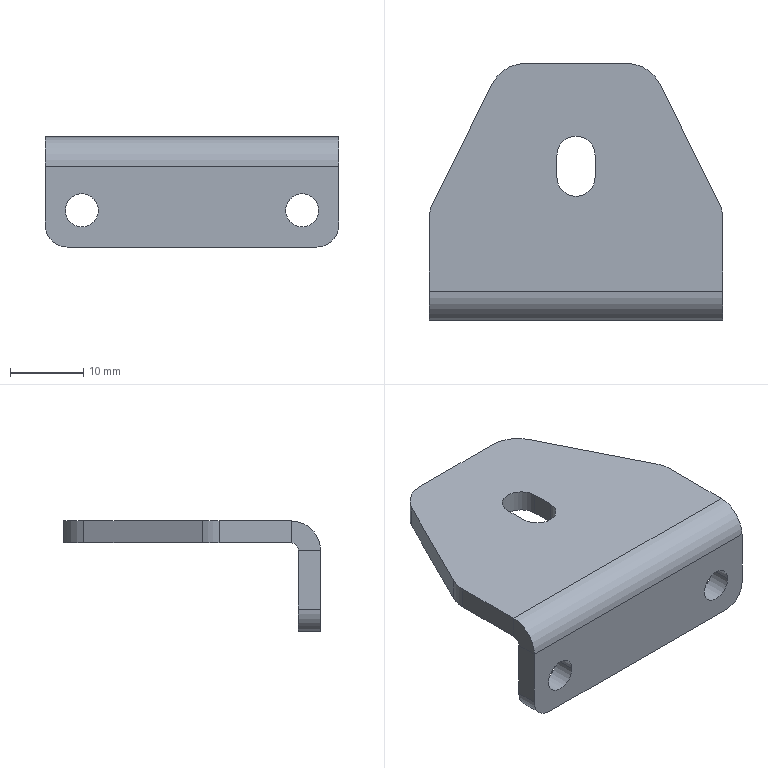Component | SolidWorks | QX1-08-BJAdapterBracket-1 | 1 solid | 30 faces | box 40 x 35 x 15 mm | volume 4683 mm3 | plane 16 | cylinder 14 | commonest cylinder face diameters 4.5 x4 10 x4 6 x2 5.203 x2 2 x1 8 x1 | material Q235
STEP:
#1=COLOUR_RGB('',0.7922,0.8196,0.9333);
#2=FILL_AREA_STYLE_COLOUR('',#1);
#3=FILL_AREA_STYLE('',(#2));
#4=SURFACE_STYLE_FILL_AREA(#3);
#5=SURFACE_SIDE_STYLE('',(#4));
#6=SURFACE_STYLE_USAGE(.BOTH.,#5);
#7=PRESENTATION_STYLE_ASSIGNMENT((#6));
#8=CARTESIAN_POINT('',(2.734,0.2002,21.801));
#9=VERTEX_POINT('',#8);
#10=CARTESIAN_POINT('',(2.557,0.2002,21.801));
#11=VERTEX_POINT('',#10);
#12=CARTESIAN_POINT('',(2.646,0.2002,21.801));
#13=DIRECTION('',(0.,1.,-0.));
#14=DIRECTION('',(-1.,0.,0.));
#15=AXIS2_PLACEMENT_3D('',#12,#13,#14);
#16=CIRCLE('',#15,0.08858);
#17=EDGE_CURVE('',#9,#11,#16,.T.);
#18=ORIENTED_EDGE('',*,*,#17,.F.);
#19=CARTESIAN_POINT('',(2.734,0.3183,21.801));
#20=VERTEX_POINT('',#19);
#21=CARTESIAN_POINT('',(2.734,0.3183,21.801));
#22=DIRECTION('',(0.,1.,-0.));
#23=VECTOR('',#22,39.37);
#24=LINE('',#21,#23);
#25=EDGE_CURVE('',#9,#20,#24,.T.);
#26=ORIENTED_EDGE('',*,*,#25,.T.);
#27=CARTESIAN_POINT('',(2.557,0.3183,21.801));
#28=VERTEX_POINT('',#27);
#29=CARTESIAN_POINT('',(2.646,0.3183,21.801));
#30=DIRECTION('',(0.,1.,-0.));
#31=DIRECTION('',(-1.,0.,0.));
#32=AXIS2_PLACEMENT_3D('',#29,#30,#31);
#33=CIRCLE('',#32,0.08858);
#34=EDGE_CURVE('',#20,#28,#33,.T.);
#35=ORIENTED_EDGE('',*,*,#34,.T.);
#36=CARTESIAN_POINT('',(2.557,0.3183,21.801));
#37=DIRECTION('',(0.,1.,-0.));
#38=VECTOR('',#37,39.37);
#39=LINE('',#36,#38);
#40=EDGE_CURVE('',#11,#28,#39,.T.);
#41=ORIENTED_EDGE('',*,*,#40,.F.);
#42=EDGE_LOOP('',(#18,#26,#35,#41));
#43=FACE_OUTER_BOUND('',#42,.T.);
#44=CARTESIAN_POINT('',(2.646,0.3183,21.801));
#45=DIRECTION('',(0.,1.,-0.));
#46=DIRECTION('',(-1.,0.,0.));
#47=AXIS2_PLACEMENT_3D('',#44,#45,#46);
#48=CYLINDRICAL_SURFACE('',#47,0.08858);
#49=ADVANCED_FACE('',(#43),#48,.F.);
#50=CARTESIAN_POINT('',(1.553,0.2002,21.801));
#51=VERTEX_POINT('',#50);
#52=CARTESIAN_POINT('',(1.376,0.2002,21.801));
#53=VERTEX_POINT('',#52);
#54=CARTESIAN_POINT('',(1.465,0.2002,21.801));
#55=DIRECTION('',(0.,1.,-0.));
#56=DIRECTION('',(-1.,0.,0.));
#57=AXIS2_PLACEMENT_3D('',#54,#55,#56);
#58=CIRCLE('',#57,0.08858);
#59=EDGE_CURVE('',#51,#53,#58,.T.);
#60=ORIENTED_EDGE('',*,*,#59,.F.);
#61=CARTESIAN_POINT('',(1.553,0.3183,21.801));
#62=VERTEX_POINT('',#61);
#63=CARTESIAN_POINT('',(1.553,0.3183,21.801));
#64=DIRECTION('',(0.,1.,-0.));
#65=VECTOR('',#64,39.37);
#66=LINE('',#63,#65);
#67=EDGE_CURVE('',#51,#62,#66,.T.);
#68=ORIENTED_EDGE('',*,*,#67,.T.);
#69=CARTESIAN_POINT('',(1.376,0.3183,21.801));
#70=VERTEX_POINT('',#69);
#71=CARTESIAN_POINT('',(1.465,0.3183,21.801));
#72=DIRECTION('',(0.,1.,-0.));
#73=DIRECTION('',(-1.,0.,0.));
#74=AXIS2_PLACEMENT_3D('',#71,#72,#73);
#75=CIRCLE('',#74,0.08858);
#76=EDGE_CURVE('',#62,#70,#75,.T.);
#77=ORIENTED_EDGE('',*,*,#76,.T.);
#78=CARTESIAN_POINT('',(1.376,0.3183,21.801));
#79=DIRECTION('',(0.,1.,-0.));
#80=VECTOR('',#79,39.37);
#81=LINE('',#78,#80);
#82=EDGE_CURVE('',#53,#70,#81,.T.);
#83=ORIENTED_EDGE('',*,*,#82,.F.);
#84=EDGE_LOOP('',(#60,#68,#77,#83));
#85=FACE_OUTER_BOUND('',#84,.T.);
#86=CARTESIAN_POINT('',(1.465,0.3183,21.801));
#87=DIRECTION('',(0.,1.,-0.));
#88=DIRECTION('',(-1.,0.,0.));
#89=AXIS2_PLACEMENT_3D('',#86,#87,#88);
#90=CYLINDRICAL_SURFACE('',#89,0.08858);
#91=ADVANCED_FACE('',(#85),#90,.F.);
#92=CARTESIAN_POINT('',(2.158,0.9679,22.195));
#93=VERTEX_POINT('',#92);
#94=CARTESIAN_POINT('',(1.953,0.9679,22.195));
#95=VERTEX_POINT('',#94);
#96=CARTESIAN_POINT('',(2.055,0.9679,22.195));
#97=DIRECTION('',(-0.,-0.,-1.));
#98=DIRECTION('',(-1.,0.,0.));
#99=AXIS2_PLACEMENT_3D('',#96,#97,#98);
#100=CIRCLE('',#99,0.1024);
#101=EDGE_CURVE('',#93,#95,#100,.T.);
#102=ORIENTED_EDGE('',*,*,#101,.T.);
#103=CARTESIAN_POINT('',(1.953,1.086,22.195));
#104=VERTEX_POINT('',#103);
#105=CARTESIAN_POINT('',(1.953,0.2002,22.195));
#106=DIRECTION('',(0.,1.,-0.));
#107=VECTOR('',#106,39.37);
#108=LINE('',#105,#107);
#109=EDGE_CURVE('',#95,#104,#108,.T.);
#110=ORIENTED_EDGE('',*,*,#109,.T.);
#111=CARTESIAN_POINT('',(2.158,1.086,22.195));
#112=VERTEX_POINT('',#111);
#113=CARTESIAN_POINT('',(2.055,1.086,22.195));
#114=DIRECTION('',(-0.,-0.,-1.));
#115=DIRECTION('',(-1.,0.,0.));
#116=AXIS2_PLACEMENT_3D('',#113,#114,#115);
#117=CIRCLE('',#116,0.1024);
#118=EDGE_CURVE('',#104,#112,#117,.T.);
#119=ORIENTED_EDGE('',*,*,#118,.T.);
#120=CARTESIAN_POINT('',(2.158,0.2002,22.195));
#121=DIRECTION('',(0.,1.,-0.));
#122=VECTOR('',#121,39.37);
#123=LINE('',#120,#122);
#124=EDGE_CURVE('',#93,#112,#123,.T.);
#125=ORIENTED_EDGE('',*,*,#124,.F.);
#126=EDGE_LOOP('',(#102,#110,#119,#125));
#127=FACE_BOUND('',#126,.T.);
#128=CARTESIAN_POINT('',(1.289,0.8323,22.195));
#129=VERTEX_POINT('',#128);
#130=CARTESIAN_POINT('',(1.607,1.469,22.195));
#131=VERTEX_POINT('',#130);
#132=CARTESIAN_POINT('',(1.268,0.7907,22.195));
#133=DIRECTION('',(0.4472,0.8944,-0.));
#134=VECTOR('',#133,39.37);
#135=LINE('',#132,#134);
#136=EDGE_CURVE('',#129,#131,#135,.T.);
#137=ORIENTED_EDGE('',*,*,#136,.F.);
#138=CARTESIAN_POINT('',(1.268,0.7442,22.195));
#139=VERTEX_POINT('',#138);
#140=CARTESIAN_POINT('',(1.465,0.7442,22.195));
#141=DIRECTION('',(0.,0.,1.));
#142=DIRECTION('',(-1.,0.,0.));
#143=AXIS2_PLACEMENT_3D('',#140,#141,#142);
#144=CIRCLE('',#143,0.1969);
#145=EDGE_CURVE('',#129,#139,#144,.T.);
#146=ORIENTED_EDGE('',*,*,#145,.T.);
#147=CARTESIAN_POINT('',(1.268,0.3576,22.195));
#148=VERTEX_POINT('',#147);
#149=CARTESIAN_POINT('',(1.268,0.2002,22.195));
#150=DIRECTION('',(0.,1.,-0.));
#151=VECTOR('',#150,39.37);
#152=LINE('',#149,#151);
#153=EDGE_CURVE('',#148,#139,#152,.T.);
#154=ORIENTED_EDGE('',*,*,#153,.F.);
#155=CARTESIAN_POINT('',(2.843,0.3576,22.195));
#156=VERTEX_POINT('',#155);
#157=CARTESIAN_POINT('',(1.268,0.3576,22.195));
#158=DIRECTION('',(1.,-0.,-0.));
#159=VECTOR('',#158,39.37);
#160=LINE('',#157,#159);
#161=EDGE_CURVE('',#148,#156,#160,.T.);
#162=ORIENTED_EDGE('',*,*,#161,.T.);
#163=CARTESIAN_POINT('',(2.843,0.7442,22.195));
#164=VERTEX_POINT('',#163);
#165=CARTESIAN_POINT('',(2.843,0.2002,22.195));
#166=DIRECTION('',(0.,1.,-0.));
#167=VECTOR('',#166,39.37);
#168=LINE('',#165,#167);
#169=EDGE_CURVE('',#156,#164,#168,.T.);
#170=ORIENTED_EDGE('',*,*,#169,.T.);
#171=CARTESIAN_POINT('',(2.822,0.8323,22.195));
#172=VERTEX_POINT('',#171);
#173=CARTESIAN_POINT('',(2.646,0.7442,22.195));
#174=DIRECTION('',(0.,0.,1.));
#175=DIRECTION('',(-1.,0.,0.));
#176=AXIS2_PLACEMENT_3D('',#173,#174,#175);
#177=CIRCLE('',#176,0.1969);
#178=EDGE_CURVE('',#164,#172,#177,.T.);
#179=ORIENTED_EDGE('',*,*,#178,.T.);
#180=CARTESIAN_POINT('',(2.503,1.469,22.195));
#181=VERTEX_POINT('',#180);
#182=CARTESIAN_POINT('',(2.843,0.7907,22.195));
#183=DIRECTION('',(-0.4472,0.8944,0.));
#184=VECTOR('',#183,39.37);
#185=LINE('',#182,#184);
#186=EDGE_CURVE('',#172,#181,#185,.T.);
#187=ORIENTED_EDGE('',*,*,#186,.T.);
#188=CARTESIAN_POINT('',(2.327,1.578,22.195));
#189=VERTEX_POINT('',#188);
#190=CARTESIAN_POINT('',(2.327,1.381,22.195));
#191=DIRECTION('',(0.,0.,1.));
#192=DIRECTION('',(-1.,0.,0.));
#193=AXIS2_PLACEMENT_3D('',#190,#191,#192);
#194=CIRCLE('',#193,0.1969);
#195=EDGE_CURVE('',#181,#189,#194,.T.);
#196=ORIENTED_EDGE('',*,*,#195,.T.);
#197=CARTESIAN_POINT('',(1.783,1.578,22.195));
#198=VERTEX_POINT('',#197);
#199=CARTESIAN_POINT('',(1.268,1.578,22.195));
#200=DIRECTION('',(1.,-0.,-0.));
#201=VECTOR('',#200,39.37);
#202=LINE('',#199,#201);
#203=EDGE_CURVE('',#198,#189,#202,.T.);
#204=ORIENTED_EDGE('',*,*,#203,.F.);
#205=CARTESIAN_POINT('',(1.783,1.381,22.195));
#206=DIRECTION('',(0.,0.,1.));
#207=DIRECTION('',(-1.,0.,0.));
#208=AXIS2_PLACEMENT_3D('',#205,#206,#207);
#209=CIRCLE('',#208,0.1969);
#210=EDGE_CURVE('',#198,#131,#209,.T.);
#211=ORIENTED_EDGE('',*,*,#210,.T.);
#212=EDGE_LOOP('',(#137,#146,#154,#162,#170,#179,#187,#196,#204,#211));
#213=FACE_OUTER_BOUND('',#212,.T.);
#214=CARTESIAN_POINT('',(1.268,0.2002,22.195));
#215=DIRECTION('',(-0.,-0.,-1.));
#216=DIRECTION('',(-1.,0.,0.));
#217=AXIS2_PLACEMENT_3D('',#214,#215,#216);
#218=PLANE('',#217);
#219=ADVANCED_FACE('',(#127,#213),#218,.F.);
#220=CARTESIAN_POINT('',(1.783,1.578,22.077));
#221=VERTEX_POINT('',#220);
#222=CARTESIAN_POINT('',(2.327,1.578,22.077));
#223=VERTEX_POINT('',#222);
#224=CARTESIAN_POINT('',(1.268,1.578,22.077));
#225=DIRECTION('',(1.,-0.,-0.));
#226=VECTOR('',#225,39.37);
#227=LINE('',#224,#226);
#228=EDGE_CURVE('',#221,#223,#227,.T.);
#229=ORIENTED_EDGE('',*,*,#228,.F.);
#230=CARTESIAN_POINT('',(1.783,1.578,22.077));
#231=DIRECTION('',(0.,0.,1.));
#232=VECTOR('',#231,39.37);
#233=LINE('',#230,#232);
#234=EDGE_CURVE('',#221,#198,#233,.T.);
#235=ORIENTED_EDGE('',*,*,#234,.T.);
#236=ORIENTED_EDGE('',*,*,#203,.T.);
#237=CARTESIAN_POINT('',(2.327,1.578,22.077));
#238=DIRECTION('',(-0.,-0.,-1.));
#239=VECTOR('',#238,39.37);
#240=LINE('',#237,#239);
#241=EDGE_CURVE('',#189,#223,#240,.T.);
#242=ORIENTED_EDGE('',*,*,#241,.T.);
#243=EDGE_LOOP('',(#229,#235,#236,#242));
#244=FACE_OUTER_BOUND('',#243,.T.);
#245=CARTESIAN_POINT('',(1.268,1.578,22.077));
#246=DIRECTION('',(0.,1.,-0.));
#247=DIRECTION('',(-1.,0.,0.));
#248=AXIS2_PLACEMENT_3D('',#245,#246,#247);
#249=PLANE('',#248);
#250=ADVANCED_FACE('',(#244),#249,.T.);
#251=CARTESIAN_POINT('',(1.953,0.9679,22.077));
#252=VERTEX_POINT('',#251);
#253=CARTESIAN_POINT('',(1.953,1.086,22.077));
#254=VERTEX_POINT('',#253);
#255=CARTESIAN_POINT('',(1.953,0.9679,22.077));
#256=DIRECTION('',(0.,1.,-0.));
#257=VECTOR('',#256,39.37);
#258=LINE('',#255,#257);
#259=EDGE_CURVE('',#252,#254,#258,.T.);
#260=ORIENTED_EDGE('',*,*,#259,.F.);
#261=CARTESIAN_POINT('',(2.158,0.9679,22.077));
#262=VERTEX_POINT('',#261);
#263=CARTESIAN_POINT('',(2.055,0.9679,22.077));
#264=DIRECTION('',(-0.,-0.,-1.));
#265=DIRECTION('',(-1.,0.,0.));
#266=AXIS2_PLACEMENT_3D('',#263,#264,#265);
#267=CIRCLE('',#266,0.1024);
#268=EDGE_CURVE('',#262,#252,#267,.T.);
#269=ORIENTED_EDGE('',*,*,#268,.F.);
#270=CARTESIAN_POINT('',(2.158,1.086,22.077));
#271=VERTEX_POINT('',#270);
#272=CARTESIAN_POINT('',(2.158,0.9679,22.077));
#273=DIRECTION('',(0.,1.,-0.));
#274=VECTOR('',#273,39.37);
#275=LINE('',#272,#274);
#276=EDGE_CURVE('',#262,#271,#275,.T.);
#277=ORIENTED_EDGE('',*,*,#276,.T.);
#278=CARTESIAN_POINT('',(2.055,1.086,22.077));
#279=DIRECTION('',(-0.,-0.,-1.));
#280=DIRECTION('',(-1.,0.,0.));
#281=AXIS2_PLACEMENT_3D('',#278,#279,#280);
#282=CIRCLE('',#281,0.1024);
#283=EDGE_CURVE('',#254,#271,#282,.T.);
#284=ORIENTED_EDGE('',*,*,#283,.F.);
#285=EDGE_LOOP('',(#260,#269,#277,#284));
#286=FACE_BOUND('',#285,.T.);
#287=CARTESIAN_POINT('',(1.268,0.3576,22.077));
#288=VERTEX_POINT('',#287);
#289=CARTESIAN_POINT('',(1.268,0.7442,22.077));
#290=VERTEX_POINT('',#289);
#291=CARTESIAN_POINT('',(1.268,0.2002,22.077));
#292=DIRECTION('',(0.,1.,-0.));
#293=VECTOR('',#292,39.37);
#294=LINE('',#291,#293);
#295=EDGE_CURVE('',#288,#290,#294,.T.);
#296=ORIENTED_EDGE('',*,*,#295,.T.);
#297=CARTESIAN_POINT('',(1.289,0.8323,22.077));
#298=VERTEX_POINT('',#297);
#299=CARTESIAN_POINT('',(1.465,0.7442,22.077));
#300=DIRECTION('',(-0.,-0.,-1.));
#301=DIRECTION('',(-1.,0.,0.));
#302=AXIS2_PLACEMENT_3D('',#299,#300,#301);
#303=CIRCLE('',#302,0.1969);
#304=EDGE_CURVE('',#290,#298,#303,.T.);
#305=ORIENTED_EDGE('',*,*,#304,.T.);
#306=CARTESIAN_POINT('',(1.607,1.469,22.077));
#307=VERTEX_POINT('',#306);
#308=CARTESIAN_POINT('',(1.268,0.7907,22.077));
#309=DIRECTION('',(0.4472,0.8944,-0.));
#310=VECTOR('',#309,39.37);
#311=LINE('',#308,#310);
#312=EDGE_CURVE('',#298,#307,#311,.T.);
#313=ORIENTED_EDGE('',*,*,#312,.T.);
#314=CARTESIAN_POINT('',(1.783,1.381,22.077));
#315=DIRECTION('',(-0.,-0.,-1.));
#316=DIRECTION('',(-1.,0.,0.));
#317=AXIS2_PLACEMENT_3D('',#314,#315,#316);
#318=CIRCLE('',#317,0.1969);
#319=EDGE_CURVE('',#307,#221,#318,.T.);
#320=ORIENTED_EDGE('',*,*,#319,.T.);
#321=ORIENTED_EDGE('',*,*,#228,.T.);
#322=CARTESIAN_POINT('',(2.503,1.469,22.077));
#323=VERTEX_POINT('',#322);
#324=CARTESIAN_POINT('',(2.327,1.381,22.077));
#325=DIRECTION('',(-0.,-0.,-1.));
#326=DIRECTION('',(-1.,0.,0.));
#327=AXIS2_PLACEMENT_3D('',#324,#325,#326);
#328=CIRCLE('',#327,0.1969);
#329=EDGE_CURVE('',#223,#323,#328,.T.);
#330=ORIENTED_EDGE('',*,*,#329,.T.);
#331=CARTESIAN_POINT('',(2.822,0.8323,22.077));
#332=VERTEX_POINT('',#331);
#333=CARTESIAN_POINT('',(2.843,0.7907,22.077));
#334=DIRECTION('',(-0.4472,0.8944,0.));
#335=VECTOR('',#334,39.37);
#336=LINE('',#333,#335);
#337=EDGE_CURVE('',#332,#323,#336,.T.);
#338=ORIENTED_EDGE('',*,*,#337,.F.);
#339=CARTESIAN_POINT('',(2.843,0.7442,22.077));
#340=VERTEX_POINT('',#339);
#341=CARTESIAN_POINT('',(2.646,0.7442,22.077));
#342=DIRECTION('',(-0.,-0.,-1.));
#343=DIRECTION('',(-1.,0.,0.));
#344=AXIS2_PLACEMENT_3D('',#341,#342,#343);
#345=CIRCLE('',#344,0.1969);
#346=EDGE_CURVE('',#332,#340,#345,.T.);
#347=ORIENTED_EDGE('',*,*,#346,.T.);
#348=CARTESIAN_POINT('',(2.843,0.3576,22.077));
#349=VERTEX_POINT('',#348);
#350=CARTESIAN_POINT('',(2.843,0.2002,22.077));
#351=DIRECTION('',(0.,1.,-0.));
#352=VECTOR('',#351,39.37);
#353=LINE('',#350,#352);
#354=EDGE_CURVE('',#349,#340,#353,.T.);
#355=ORIENTED_EDGE('',*,*,#354,.F.);
#356=CARTESIAN_POINT('',(1.268,0.3576,22.077));
#357=DIRECTION('',(1.,-0.,-0.));
#358=VECTOR('',#357,39.37);
#359=LINE('',#356,#358);
#360=EDGE_CURVE('',#288,#349,#359,.T.);
#361=ORIENTED_EDGE('',*,*,#360,.F.);
#362=EDGE_LOOP('',(#296,#305,#313,#320,#321,#330,#338,#347,#355,#361));
#363=FACE_OUTER_BOUND('',#362,.T.);
#364=CARTESIAN_POINT('',(1.268,0.2002,22.077));
#365=DIRECTION('',(-0.,-0.,-1.));
#366=DIRECTION('',(-1.,0.,0.));
#367=AXIS2_PLACEMENT_3D('',#364,#365,#366);
#368=PLANE('',#367);
#369=ADVANCED_FACE('',(#286,#363),#368,.T.);
#370=ORIENTED_EDGE('',*,*,#153,.T.);
#371=CARTESIAN_POINT('',(1.268,0.7442,22.037));
#372=DIRECTION('',(-0.,-0.,-1.));
#373=VECTOR('',#372,39.37);
#374=LINE('',#371,#373);
#375=EDGE_CURVE('',#139,#290,#374,.T.);
#376=ORIENTED_EDGE('',*,*,#375,.T.);
#377=ORIENTED_EDGE('',*,*,#295,.F.);
#378=CARTESIAN_POINT('',(1.268,0.3576,22.077));
#379=DIRECTION('',(0.,0.,1.));
#380=VECTOR('',#379,39.37);
#381=LINE('',#378,#380);
#382=EDGE_CURVE('',#288,#148,#381,.T.);
#383=ORIENTED_EDGE('',*,*,#382,.T.);
#384=EDGE_LOOP('',(#370,#376,#377,#383));
#385=FACE_OUTER_BOUND('',#384,.T.);
#386=CARTESIAN_POINT('',(1.268,0.3576,22.037));
#387=DIRECTION('',(-1.,0.,0.));
#388=DIRECTION('',(0.,0.,1.));
#389=AXIS2_PLACEMENT_3D('',#386,#387,#388);
#390=PLANE('',#389);
#391=ADVANCED_FACE('',(#385),#390,.T.);
#392=CARTESIAN_POINT('',(1.268,0.2002,22.037));
#393=VERTEX_POINT('',#392);
#394=CARTESIAN_POINT('',(1.268,0.3183,22.037));
#395=VERTEX_POINT('',#394);
#396=CARTESIAN_POINT('',(1.268,0.2002,22.037));
#397=DIRECTION('',(0.,1.,-0.));
#398=VECTOR('',#397,39.37);
#399=LINE('',#396,#398);
#400=EDGE_CURVE('',#393,#395,#399,.T.);
#401=ORIENTED_EDGE('',*,*,#400,.F.);
#402=CARTESIAN_POINT('',(1.268,0.3576,22.037));
#403=DIRECTION('',(-1.,0.,0.));
#404=DIRECTION('',(-0.,0.,-1.));
#405=AXIS2_PLACEMENT_3D('',#402,#403,#404);
#406=CIRCLE('',#405,0.1575);
#407=EDGE_CURVE('',#393,#148,#406,.T.);
#408=ORIENTED_EDGE('',*,*,#407,.T.);
#409=ORIENTED_EDGE('',*,*,#382,.F.);
#410=CARTESIAN_POINT('',(1.268,0.3576,22.037));
#411=DIRECTION('',(-1.,0.,0.));
#412=DIRECTION('',(0.,0.,1.));
#413=AXIS2_PLACEMENT_3D('',#410,#411,#412);
#414=CIRCLE('',#413,0.03937);
#415=EDGE_CURVE('',#395,#288,#414,.T.);
#416=ORIENTED_EDGE('',*,*,#415,.F.);
#417=EDGE_LOOP('',(#401,#408,#409,#416));
#418=FACE_OUTER_BOUND('',#417,.T.);
#419=CARTESIAN_POINT('',(1.268,0.2002,22.037));
#420=DIRECTION('',(-1.,0.,0.));
#421=DIRECTION('',(0.,0.,1.));
#422=AXIS2_PLACEMENT_3D('',#419,#420,#421);
#423=PLANE('',#422);
#424=ADVANCED_FACE('',(#418),#423,.T.);
#425=CARTESIAN_POINT('',(1.268,0.3183,21.722));
#426=VERTEX_POINT('',#425);
#427=CARTESIAN_POINT('',(1.268,0.3183,21.604));
#428=DIRECTION('',(0.,0.,1.));
#429=VECTOR('',#428,39.37);
#430=LINE('',#427,#429);
#431=EDGE_CURVE('',#426,#395,#430,.T.);
#432=ORIENTED_EDGE('',*,*,#431,.F.);
#433=CARTESIAN_POINT('',(1.268,0.2002,21.722));
#434=VERTEX_POINT('',#433);
#435=CARTESIAN_POINT('',(1.268,0.3576,21.722));
#436=DIRECTION('',(-0.,-1.,0.));
#437=VECTOR('',#436,39.37);
#438=LINE('',#435,#437);
#439=EDGE_CURVE('',#426,#434,#438,.T.);
#440=ORIENTED_EDGE('',*,*,#439,.T.);
#441=CARTESIAN_POINT('',(1.268,0.2002,21.604));
#442=DIRECTION('',(0.,0.,1.));
#443=VECTOR('',#442,39.37);
#444=LINE('',#441,#443);
#445=EDGE_CURVE('',#434,#393,#444,.T.);
#446=ORIENTED_EDGE('',*,*,#445,.T.);
#447=ORIENTED_EDGE('',*,*,#400,.T.);
#448=EDGE_LOOP('',(#432,#440,#446,#447));
#449=FACE_OUTER_BOUND('',#448,.T.);
#450=CARTESIAN_POINT('',(1.268,0.3576,22.077));
#451=DIRECTION('',(-1.,0.,0.));
#452=DIRECTION('',(0.,0.,1.));
#453=AXIS2_PLACEMENT_3D('',#450,#451,#452);
#454=PLANE('',#453);
#455=ADVANCED_FACE('',(#449),#454,.T.);
#456=CARTESIAN_POINT('',(2.843,0.3576,22.195));
#457=DIRECTION('',(-0.,-0.,-1.));
#458=VECTOR('',#457,39.37);
#459=LINE('',#456,#458);
#460=EDGE_CURVE('',#156,#349,#459,.T.);
#461=ORIENTED_EDGE('',*,*,#460,.F.);
#462=CARTESIAN_POINT('',(2.843,0.2002,22.037));
#463=VERTEX_POINT('',#462);
#464=CARTESIAN_POINT('',(2.843,0.3576,22.037));
#465=DIRECTION('',(-1.,0.,0.));
#466=DIRECTION('',(0.,0.,-1.));
#467=AXIS2_PLACEMENT_3D('',#464,#465,#466);
#468=CIRCLE('',#467,0.1575);
#469=EDGE_CURVE('',#463,#156,#468,.T.);
#470=ORIENTED_EDGE('',*,*,#469,.F.);
#471=CARTESIAN_POINT('',(2.843,0.3183,22.037));
#472=VERTEX_POINT('',#471);
#473=CARTESIAN_POINT('',(2.843,0.3183,22.037));
#474=DIRECTION('',(-0.,-1.,0.));
#475=VECTOR('',#474,39.37);
#476=LINE('',#473,#475);
#477=EDGE_CURVE('',#472,#463,#476,.T.);
#478=ORIENTED_EDGE('',*,*,#477,.F.);
#479=CARTESIAN_POINT('',(2.843,0.3576,22.037));
#480=DIRECTION('',(-1.,0.,0.));
#481=DIRECTION('',(0.,0.,1.));
#482=AXIS2_PLACEMENT_3D('',#479,#480,#481);
#483=CIRCLE('',#482,0.03937);
#484=EDGE_CURVE('',#472,#349,#483,.T.);
#485=ORIENTED_EDGE('',*,*,#484,.T.);
#486=EDGE_LOOP('',(#461,#470,#478,#485));
#487=FACE_OUTER_BOUND('',#486,.T.);
#488=CARTESIAN_POINT('',(2.843,0.3576,22.195));
#489=DIRECTION('',(1.,-0.,-0.));
#490=DIRECTION('',(-0.,-0.,-1.));
#491=AXIS2_PLACEMENT_3D('',#488,#489,#490);
#492=PLANE('',#491);
#493=ADVANCED_FACE('',(#487),#492,.T.);
#494=ORIENTED_EDGE('',*,*,#354,.T.);
#495=CARTESIAN_POINT('',(2.843,0.7442,22.195));
#496=DIRECTION('',(0.,0.,1.));
#497=VECTOR('',#496,39.37);
#498=LINE('',#495,#497);
#499=EDGE_CURVE('',#340,#164,#498,.T.);
#500=ORIENTED_EDGE('',*,*,#499,.T.);
#501=ORIENTED_EDGE('',*,*,#169,.F.);
#502=ORIENTED_EDGE('',*,*,#460,.T.);
#503=EDGE_LOOP('',(#494,#500,#501,#502));
#504=FACE_OUTER_BOUND('',#503,.T.);
#505=CARTESIAN_POINT('',(2.843,0.3183,22.037));
#506=DIRECTION('',(1.,-0.,-0.));
#507=DIRECTION('',(-0.,-0.,-1.));
#508=AXIS2_PLACEMENT_3D('',#505,#506,#507);
#509=PLANE('',#508);
#510=ADVANCED_FACE('',(#504),#509,.T.);
#511=ORIENTED_EDGE('',*,*,#484,.F.);
#512=CARTESIAN_POINT('',(1.268,0.3183,22.037));
#513=DIRECTION('',(1.,-0.,-0.));
#514=VECTOR('',#513,39.37);
#515=LINE('',#512,#514);
#516=EDGE_CURVE('',#395,#472,#515,.T.);
#517=ORIENTED_EDGE('',*,*,#516,.F.);
#518=ORIENTED_EDGE('',*,*,#415,.T.);
#519=ORIENTED_EDGE('',*,*,#360,.T.);
#520=EDGE_LOOP('',(#511,#517,#518,#519));
#521=FACE_OUTER_BOUND('',#520,.T.);
#522=CARTESIAN_POINT('',(1.268,0.3576,22.037));
#523=DIRECTION('',(1.,-0.,-0.));
#524=DIRECTION('',(0.,0.,-1.));
#525=AXIS2_PLACEMENT_3D('',#522,#523,#524);
#526=CYLINDRICAL_SURFACE('',#525,0.03937);
#527=ADVANCED_FACE('',(#521),#526,.F.);
#528=CARTESIAN_POINT('',(2.646,0.3183,21.801));
#529=DIRECTION('',(0.,1.,-0.));
#530=DIRECTION('',(-1.,0.,0.));
#531=AXIS2_PLACEMENT_3D('',#528,#529,#530);
#532=CIRCLE('',#531,0.08858);
#533=EDGE_CURVE('',#28,#20,#532,.T.);
#534=ORIENTED_EDGE('',*,*,#533,.F.);
#535=ORIENTED_EDGE('',*,*,#34,.F.);
#536=EDGE_LOOP('',(#534,#535));
#537=FACE_BOUND('',#536,.T.);
#538=CARTESIAN_POINT('',(1.465,0.3183,21.801));
#539=DIRECTION('',(0.,1.,-0.));
#540=DIRECTION('',(-1.,0.,0.));
#541=AXIS2_PLACEMENT_3D('',#538,#539,#540);
#542=CIRCLE('',#541,0.08858);
#543=EDGE_CURVE('',#70,#62,#542,.T.);
#544=ORIENTED_EDGE('',*,*,#543,.F.);
#545=ORIENTED_EDGE('',*,*,#76,.F.);
#546=EDGE_LOOP('',(#544,#545));
#547=FACE_BOUND('',#546,.T.);
#548=CARTESIAN_POINT('',(1.386,0.3183,21.604));
#549=VERTEX_POINT('',#548);
#550=CARTESIAN_POINT('',(2.725,0.3183,21.604));
#551=VERTEX_POINT('',#550);
#552=CARTESIAN_POINT('',(1.268,0.3183,21.604));
#553=DIRECTION('',(1.,-0.,-0.));
#554=VECTOR('',#553,39.37);
#555=LINE('',#552,#554);
#556=EDGE_CURVE('',#549,#551,#555,.T.);
#557=ORIENTED_EDGE('',*,*,#556,.F.);
#558=CARTESIAN_POINT('',(1.386,0.3183,21.722));
#559=DIRECTION('',(0.,1.,-0.));
#560=DIRECTION('',(-1.,0.,0.));
#561=AXIS2_PLACEMENT_3D('',#558,#559,#560);
#562=CIRCLE('',#561,0.1181);
#563=EDGE_CURVE('',#549,#426,#562,.T.);
#564=ORIENTED_EDGE('',*,*,#563,.T.);
#565=ORIENTED_EDGE('',*,*,#431,.T.);
#566=ORIENTED_EDGE('',*,*,#516,.T.);
#567=CARTESIAN_POINT('',(2.843,0.3183,21.722));
#568=VERTEX_POINT('',#567);
#569=CARTESIAN_POINT('',(2.843,0.3183,21.604));
#570=DIRECTION('',(0.,0.,1.));
#571=VECTOR('',#570,39.37);
#572=LINE('',#569,#571);
#573=EDGE_CURVE('',#568,#472,#572,.T.);
#574=ORIENTED_EDGE('',*,*,#573,.F.);
#575=CARTESIAN_POINT('',(2.725,0.3183,21.722));
#576=DIRECTION('',(0.,1.,-0.));
#577=DIRECTION('',(-1.,0.,0.));
#578=AXIS2_PLACEMENT_3D('',#575,#576,#577);
#579=CIRCLE('',#578,0.1181);
#580=EDGE_CURVE('',#568,#551,#579,.T.);
#581=ORIENTED_EDGE('',*,*,#580,.T.);
#582=EDGE_LOOP('',(#557,#564,#565,#566,#574,#581));
#583=FACE_OUTER_BOUND('',#582,.T.);
#584=CARTESIAN_POINT('',(1.268,0.3183,21.604));
#585=DIRECTION('',(0.,1.,-0.));
#586=DIRECTION('',(-1.,0.,0.));
#587=AXIS2_PLACEMENT_3D('',#584,#585,#586);
#588=PLANE('',#587);
#589=ADVANCED_FACE('',(#537,#547,#583),#588,.T.);
#590=CARTESIAN_POINT('',(1.386,0.2002,21.604));
#591=VERTEX_POINT('',#590);
#592=CARTESIAN_POINT('',(2.725,0.2002,21.604));
#593=VERTEX_POINT('',#592);
#594=CARTESIAN_POINT('',(1.268,0.2002,21.604));
#595=DIRECTION('',(1.,-0.,-0.));
#596=VECTOR('',#595,39.37);
#597=LINE('',#594,#596);
#598=EDGE_CURVE('',#591,#593,#597,.T.);
#599=ORIENTED_EDGE('',*,*,#598,.F.);
#600=CARTESIAN_POINT('',(1.386,0.2002,21.604));
#601=DIRECTION('',(0.,1.,-0.));
#602=VECTOR('',#601,39.37);
#603=LINE('',#600,#602);
#604=EDGE_CURVE('',#591,#549,#603,.T.);
#605=ORIENTED_EDGE('',*,*,#604,.T.);
#606=ORIENTED_EDGE('',*,*,#556,.T.);
#607=CARTESIAN_POINT('',(2.725,0.2002,21.604));
#608=DIRECTION('',(-0.,-1.,0.));
#609=VECTOR('',#608,39.37);
#610=LINE('',#607,#609);
#611=EDGE_CURVE('',#551,#593,#610,.T.);
#612=ORIENTED_EDGE('',*,*,#611,.T.);
#613=EDGE_LOOP('',(#599,#605,#606,#612));
#614=FACE_OUTER_BOUND('',#613,.T.);
#615=CARTESIAN_POINT('',(1.268,0.2002,21.604));
#616=DIRECTION('',(-0.,-0.,-1.));
#617=DIRECTION('',(-1.,0.,0.));
#618=AXIS2_PLACEMENT_3D('',#615,#616,#617);
#619=PLANE('',#618);
#620=ADVANCED_FACE('',(#614),#619,.T.);
#621=CARTESIAN_POINT('',(2.646,0.2002,21.801));
#622=DIRECTION('',(0.,1.,-0.));
#623=DIRECTION('',(-1.,0.,0.));
#624=AXIS2_PLACEMENT_3D('',#621,#622,#623);
#625=CIRCLE('',#624,0.08858);
#626=EDGE_CURVE('',#11,#9,#625,.T.);
#627=ORIENTED_EDGE('',*,*,#626,.T.);
#628=ORIENTED_EDGE('',*,*,#17,.T.);
#629=EDGE_LOOP('',(#627,#628));
#630=FACE_BOUND('',#629,.T.);
#631=CARTESIAN_POINT('',(1.465,0.2002,21.801));
#632=DIRECTION('',(0.,1.,-0.));
#633=DIRECTION('',(-1.,0.,0.));
#634=AXIS2_PLACEMENT_3D('',#631,#632,#633);
#635=CIRCLE('',#634,0.08858);
#636=EDGE_CURVE('',#53,#51,#635,.T.);
#637=ORIENTED_EDGE('',*,*,#636,.T.);
#638=ORIENTED_EDGE('',*,*,#59,.T.);
#639=EDGE_LOOP('',(#637,#638));
#640=FACE_BOUND('',#639,.T.);
#641=ORIENTED_EDGE('',*,*,#445,.F.);
#642=CARTESIAN_POINT('',(1.386,0.2002,21.722));
#643=DIRECTION('',(-0.,-1.,0.));
#644=DIRECTION('',(-1.,0.,0.));
#645=AXIS2_PLACEMENT_3D('',#642,#643,#644);
#646=CIRCLE('',#645,0.1181);
#647=EDGE_CURVE('',#434,#591,#646,.T.);
#648=ORIENTED_EDGE('',*,*,#647,.T.);
#649=ORIENTED_EDGE('',*,*,#598,.T.);
#650=CARTESIAN_POINT('',(2.843,0.2002,21.722));
#651=VERTEX_POINT('',#650);
#652=CARTESIAN_POINT('',(2.725,0.2002,21.722));
#653=DIRECTION('',(-0.,-1.,0.));
#654=DIRECTION('',(-1.,0.,0.));
#655=AXIS2_PLACEMENT_3D('',#652,#653,#654);
#656=CIRCLE('',#655,0.1181);
#657=EDGE_CURVE('',#593,#651,#656,.T.);
#658=ORIENTED_EDGE('',*,*,#657,.T.);
#659=CARTESIAN_POINT('',(2.843,0.2002,21.604));
#660=DIRECTION('',(0.,0.,1.));
#661=VECTOR('',#660,39.37);
#662=LINE('',#659,#661);
#663=EDGE_CURVE('',#651,#463,#662,.T.);
#664=ORIENTED_EDGE('',*,*,#663,.T.);
#665=CARTESIAN_POINT('',(1.268,0.2002,22.037));
#666=DIRECTION('',(1.,-0.,-0.));
#667=VECTOR('',#666,39.37);
#668=LINE('',#665,#667);
#669=EDGE_CURVE('',#393,#463,#668,.T.);
#670=ORIENTED_EDGE('',*,*,#669,.F.);
#671=EDGE_LOOP('',(#641,#648,#649,#658,#664,#670));
#672=FACE_OUTER_BOUND('',#671,.T.);
#673=CARTESIAN_POINT('',(1.268,0.2002,21.604));
#674=DIRECTION('',(0.,1.,-0.));
#675=DIRECTION('',(-1.,0.,0.));
#676=AXIS2_PLACEMENT_3D('',#673,#674,#675);
#677=PLANE('',#676);
#678=ADVANCED_FACE('',(#630,#640,#672),#677,.F.);
#679=ORIENTED_EDGE('',*,*,#469,.T.);
#680=ORIENTED_EDGE('',*,*,#161,.F.);
#681=ORIENTED_EDGE('',*,*,#407,.F.);
#682=ORIENTED_EDGE('',*,*,#669,.T.);
#683=EDGE_LOOP('',(#679,#680,#681,#682));
#684=FACE_OUTER_BOUND('',#683,.T.);
#685=CARTESIAN_POINT('',(1.268,0.3576,22.037));
#686=DIRECTION('',(1.,-0.,-0.));
#687=DIRECTION('',(-0.,0.,-1.));
#688=AXIS2_PLACEMENT_3D('',#685,#686,#687);
#689=CYLINDRICAL_SURFACE('',#688,0.1575);
#690=ADVANCED_FACE('',(#684),#689,.T.);
#691=ORIENTED_EDGE('',*,*,#663,.F.);
#692=CARTESIAN_POINT('',(2.843,0.3183,21.722));
#693=DIRECTION('',(0.,1.,-0.));
#694=VECTOR('',#693,39.37);
#695=LINE('',#692,#694);
#696=EDGE_CURVE('',#651,#568,#695,.T.);
#697=ORIENTED_EDGE('',*,*,#696,.T.);
#698=ORIENTED_EDGE('',*,*,#573,.T.);
#699=ORIENTED_EDGE('',*,*,#477,.T.);
#700=EDGE_LOOP('',(#691,#697,#698,#699));
#701=FACE_OUTER_BOUND('',#700,.T.);
#702=CARTESIAN_POINT('',(2.843,0.3576,22.037));
#703=DIRECTION('',(-1.,0.,0.));
#704=DIRECTION('',(0.,0.,1.));
#705=AXIS2_PLACEMENT_3D('',#702,#703,#704);
#706=PLANE('',#705);
#707=ADVANCED_FACE('',(#701),#706,.F.);
#708=ORIENTED_EDGE('',*,*,#186,.F.);
#709=CARTESIAN_POINT('',(2.822,0.8323,22.077));
#710=DIRECTION('',(-0.,-0.,-1.));
#711=VECTOR('',#710,39.37);
#712=LINE('',#709,#711);
#713=EDGE_CURVE('',#172,#332,#712,.T.);
#714=ORIENTED_EDGE('',*,*,#713,.T.);
#715=ORIENTED_EDGE('',*,*,#337,.T.);
#716=CARTESIAN_POINT('',(2.503,1.469,22.195));
#717=DIRECTION('',(0.,0.,1.));
#718=VECTOR('',#717,39.37);
#719=LINE('',#716,#718);
#720=EDGE_CURVE('',#323,#181,#719,.T.);
#721=ORIENTED_EDGE('',*,*,#720,.T.);
#722=EDGE_LOOP('',(#708,#714,#715,#721));
#723=FACE_OUTER_BOUND('',#722,.T.);
#724=CARTESIAN_POINT('',(2.843,0.7907,22.195));
#725=DIRECTION('',(-0.8944,-0.4472,0.));
#726=DIRECTION('',(0.4472,-0.8944,-0.));
#727=AXIS2_PLACEMENT_3D('',#724,#725,#726);
#728=PLANE('',#727);
#729=ADVANCED_FACE('',(#723),#728,.F.);
#730=ORIENTED_EDGE('',*,*,#312,.F.);
#731=CARTESIAN_POINT('',(1.289,0.8323,22.195));
#732=DIRECTION('',(0.,0.,1.));
#733=VECTOR('',#732,39.37);
#734=LINE('',#731,#733);
#735=EDGE_CURVE('',#298,#129,#734,.T.);
#736=ORIENTED_EDGE('',*,*,#735,.T.);
#737=ORIENTED_EDGE('',*,*,#136,.T.);
#738=CARTESIAN_POINT('',(1.607,1.469,22.195));
#739=DIRECTION('',(-0.,-0.,-1.));
#740=VECTOR('',#739,39.37);
#741=LINE('',#738,#740);
#742=EDGE_CURVE('',#131,#307,#741,.T.);
#743=ORIENTED_EDGE('',*,*,#742,.T.);
#744=EDGE_LOOP('',(#730,#736,#737,#743));
#745=FACE_OUTER_BOUND('',#744,.T.);
#746=CARTESIAN_POINT('',(1.268,0.7907,22.195));
#747=DIRECTION('',(-0.8944,0.4472,0.));
#748=DIRECTION('',(-0.4472,-0.8944,0.));
#749=AXIS2_PLACEMENT_3D('',#746,#747,#748);
#750=PLANE('',#749);
#751=ADVANCED_FACE('',(#745),#750,.T.);
#752=ORIENTED_EDGE('',*,*,#145,.F.);
#753=ORIENTED_EDGE('',*,*,#735,.F.);
#754=ORIENTED_EDGE('',*,*,#304,.F.);
#755=ORIENTED_EDGE('',*,*,#375,.F.);
#756=EDGE_LOOP('',(#752,#753,#754,#755));
#757=FACE_OUTER_BOUND('',#756,.T.);
#758=CARTESIAN_POINT('',(1.465,0.7442,22.037));
#759=DIRECTION('',(-0.,-0.,-1.));
#760=DIRECTION('',(-1.,0.,0.));
#761=AXIS2_PLACEMENT_3D('',#758,#759,#760);
#762=CYLINDRICAL_SURFACE('',#761,0.1969);
#763=ADVANCED_FACE('',(#757),#762,.T.);
#764=ORIENTED_EDGE('',*,*,#178,.F.);
#765=ORIENTED_EDGE('',*,*,#499,.F.);
#766=ORIENTED_EDGE('',*,*,#346,.F.);
#767=ORIENTED_EDGE('',*,*,#713,.F.);
#768=EDGE_LOOP('',(#764,#765,#766,#767));
#769=FACE_OUTER_BOUND('',#768,.T.);
#770=CARTESIAN_POINT('',(2.646,0.7442,22.195));
#771=DIRECTION('',(0.,0.,1.));
#772=DIRECTION('',(1.,0.,0.));
#773=AXIS2_PLACEMENT_3D('',#770,#771,#772);
#774=CYLINDRICAL_SURFACE('',#773,0.1969);
#775=ADVANCED_FACE('',(#769),#774,.T.);
#776=ORIENTED_EDGE('',*,*,#210,.F.);
#777=ORIENTED_EDGE('',*,*,#234,.F.);
#778=ORIENTED_EDGE('',*,*,#319,.F.);
#779=ORIENTED_EDGE('',*,*,#742,.F.);
#780=EDGE_LOOP('',(#776,#777,#778,#779));
#781=FACE_OUTER_BOUND('',#780,.T.);
#782=CARTESIAN_POINT('',(1.783,1.381,22.195));
#783=DIRECTION('',(-0.,-0.,-1.));
#784=DIRECTION('',(-1.,0.,0.));
#785=AXIS2_PLACEMENT_3D('',#782,#783,#784);
#786=CYLINDRICAL_SURFACE('',#785,0.1969);
#787=ADVANCED_FACE('',(#781),#786,.T.);
#788=ORIENTED_EDGE('',*,*,#195,.F.);
#789=ORIENTED_EDGE('',*,*,#720,.F.);
#790=ORIENTED_EDGE('',*,*,#329,.F.);
#791=ORIENTED_EDGE('',*,*,#241,.F.);
#792=EDGE_LOOP('',(#788,#789,#790,#791));
#793=FACE_OUTER_BOUND('',#792,.T.);
#794=CARTESIAN_POINT('',(2.327,1.381,22.077));
#795=DIRECTION('',(0.,0.,1.));
#796=DIRECTION('',(1.,0.,0.));
#797=AXIS2_PLACEMENT_3D('',#794,#795,#796);
#798=CYLINDRICAL_SURFACE('',#797,0.1969);
#799=ADVANCED_FACE('',(#793),#798,.T.);
#800=ORIENTED_EDGE('',*,*,#647,.F.);
#801=ORIENTED_EDGE('',*,*,#439,.F.);
#802=ORIENTED_EDGE('',*,*,#563,.F.);
#803=ORIENTED_EDGE('',*,*,#604,.F.);
#804=EDGE_LOOP('',(#800,#801,#802,#803));
#805=FACE_OUTER_BOUND('',#804,.T.);
#806=CARTESIAN_POINT('',(1.386,0.2002,21.722));
#807=DIRECTION('',(0.,1.,-0.));
#808=DIRECTION('',(-1.,0.,0.));
#809=AXIS2_PLACEMENT_3D('',#806,#807,#808);
#810=CYLINDRICAL_SURFACE('',#809,0.1181);
#811=ADVANCED_FACE('',(#805),#810,.T.);
#812=ORIENTED_EDGE('',*,*,#657,.F.);
#813=ORIENTED_EDGE('',*,*,#611,.F.);
#814=ORIENTED_EDGE('',*,*,#580,.F.);
#815=ORIENTED_EDGE('',*,*,#696,.F.);
#816=EDGE_LOOP('',(#812,#813,#814,#815));
#817=FACE_OUTER_BOUND('',#816,.T.);
#818=CARTESIAN_POINT('',(2.725,0.3576,21.722));
#819=DIRECTION('',(-0.,-1.,0.));
#820=DIRECTION('',(1.,0.,0.));
#821=AXIS2_PLACEMENT_3D('',#818,#819,#820);
#822=CYLINDRICAL_SURFACE('',#821,0.1181);
#823=ADVANCED_FACE('',(#817),#822,.T.);
#824=ORIENTED_EDGE('',*,*,#67,.F.);
#825=ORIENTED_EDGE('',*,*,#636,.F.);
#826=ORIENTED_EDGE('',*,*,#82,.T.);
#827=ORIENTED_EDGE('',*,*,#543,.T.);
#828=EDGE_LOOP('',(#824,#825,#826,#827));
#829=FACE_OUTER_BOUND('',#828,.T.);
#830=CARTESIAN_POINT('',(1.465,0.3183,21.801));
#831=DIRECTION('',(0.,1.,-0.));
#832=DIRECTION('',(-1.,0.,0.));
#833=AXIS2_PLACEMENT_3D('',#830,#831,#832);
#834=CYLINDRICAL_SURFACE('',#833,0.08858);
#835=ADVANCED_FACE('',(#829),#834,.F.);
#836=ORIENTED_EDGE('',*,*,#25,.F.);
#837=ORIENTED_EDGE('',*,*,#626,.F.);
#838=ORIENTED_EDGE('',*,*,#40,.T.);
#839=ORIENTED_EDGE('',*,*,#533,.T.);
#840=EDGE_LOOP('',(#836,#837,#838,#839));
#841=FACE_OUTER_BOUND('',#840,.T.);
#842=CARTESIAN_POINT('',(2.646,0.3183,21.801));
#843=DIRECTION('',(0.,1.,-0.));
#844=DIRECTION('',(-1.,0.,0.));
#845=AXIS2_PLACEMENT_3D('',#842,#843,#844);
#846=CYLINDRICAL_SURFACE('',#845,0.08858);
#847=ADVANCED_FACE('',(#841),#846,.F.);
#848=CARTESIAN_POINT('',(1.953,0.9679,22.47));
#849=DIRECTION('',(-0.,-0.,-1.));
#850=VECTOR('',#849,39.37);
#851=LINE('',#848,#850);
#852=EDGE_CURVE('',#95,#252,#851,.T.);
#853=ORIENTED_EDGE('',*,*,#852,.T.);
#854=ORIENTED_EDGE('',*,*,#259,.T.);
#855=CARTESIAN_POINT('',(1.953,1.086,22.47));
#856=DIRECTION('',(-0.,-0.,-1.));
#857=VECTOR('',#856,39.37);
#858=LINE('',#855,#857);
#859=EDGE_CURVE('',#104,#254,#858,.T.);
#860=ORIENTED_EDGE('',*,*,#859,.F.);
#861=ORIENTED_EDGE('',*,*,#109,.F.);
#862=EDGE_LOOP('',(#853,#854,#860,#861));
#863=FACE_OUTER_BOUND('',#862,.T.);
#864=CARTESIAN_POINT('',(1.953,0.9679,22.47));
#865=DIRECTION('',(-1.,0.,0.));
#866=DIRECTION('',(-0.,-1.,0.));
#867=AXIS2_PLACEMENT_3D('',#864,#865,#866);
#868=PLANE('',#867);
#869=ADVANCED_FACE('',(#863),#868,.F.);
#870=CARTESIAN_POINT('',(2.158,0.9679,22.47));
#871=DIRECTION('',(-0.,-0.,-1.));
#872=VECTOR('',#871,39.37);
#873=LINE('',#870,#872);
#874=EDGE_CURVE('',#93,#262,#873,.T.);
#875=ORIENTED_EDGE('',*,*,#874,.T.);
#876=ORIENTED_EDGE('',*,*,#268,.T.);
#877=ORIENTED_EDGE('',*,*,#852,.F.);
#878=ORIENTED_EDGE('',*,*,#101,.F.);
#879=EDGE_LOOP('',(#875,#876,#877,#878));
#880=FACE_OUTER_BOUND('',#879,.T.);
#881=CARTESIAN_POINT('',(2.055,0.9679,22.47));
#882=DIRECTION('',(-0.,-0.,-1.));
#883=DIRECTION('',(-1.,0.,0.));
#884=AXIS2_PLACEMENT_3D('',#881,#882,#883);
#885=CYLINDRICAL_SURFACE('',#884,0.1024);
#886=ADVANCED_FACE('',(#880),#885,.F.);
#887=ORIENTED_EDGE('',*,*,#124,.T.);
#888=CARTESIAN_POINT('',(2.158,1.086,22.47));
#889=DIRECTION('',(-0.,-0.,-1.));
#890=VECTOR('',#889,39.37);
#891=LINE('',#888,#890);
#892=EDGE_CURVE('',#112,#271,#891,.T.);
#893=ORIENTED_EDGE('',*,*,#892,.T.);
#894=ORIENTED_EDGE('',*,*,#276,.F.);
#895=ORIENTED_EDGE('',*,*,#874,.F.);
#896=EDGE_LOOP('',(#887,#893,#894,#895));
#897=FACE_OUTER_BOUND('',#896,.T.);
#898=CARTESIAN_POINT('',(2.158,0.9679,22.47));
#899=DIRECTION('',(-1.,0.,0.));
#900=DIRECTION('',(-0.,-1.,0.));
#901=AXIS2_PLACEMENT_3D('',#898,#899,#900);
#902=PLANE('',#901);
#903=ADVANCED_FACE('',(#897),#902,.T.);
#904=ORIENTED_EDGE('',*,*,#859,.T.);
#905=ORIENTED_EDGE('',*,*,#283,.T.);
#906=ORIENTED_EDGE('',*,*,#892,.F.);
#907=ORIENTED_EDGE('',*,*,#118,.F.);
#908=EDGE_LOOP('',(#904,#905,#906,#907));
#909=FACE_OUTER_BOUND('',#908,.T.);
#910=CARTESIAN_POINT('',(2.055,1.086,22.47));
#911=DIRECTION('',(-0.,-0.,-1.));
#912=DIRECTION('',(-1.,0.,0.));
#913=AXIS2_PLACEMENT_3D('',#910,#911,#912);
#914=CYLINDRICAL_SURFACE('',#913,0.1024);
#915=ADVANCED_FACE('',(#909),#914,.F.);
#916=CLOSED_SHELL('',(#49,#91,#219,#250,#369,#391,#424,#455,#493,#510,#527,#589,#620,#678,#690,#707,#729,#751,#763,#775,#787,#799,#811,#823,#835,#847,#869,#886,#903,#915));
#917=MANIFOLD_SOLID_BREP('',#916);
#918=STYLED_ITEM('',(#7),#917);
#919=PRESENTATION_LAYER_ASSIGNMENT('','',(#918));
#920=CARTESIAN_POINT('',(0.,0.,0.));
#921=DIRECTION('',(0.,0.,1.));
#922=DIRECTION('',(1.,0.,0.));
#923=AXIS2_PLACEMENT_3D('',#920,#921,#922);
#924=(LENGTH_UNIT()NAMED_UNIT(*)SI_UNIT($,.METRE.));
#925=LENGTH_MEASURE_WITH_UNIT(LENGTH_MEASURE(0.0254),#924);
#926=DIMENSIONAL_EXPONENTS(1.,0.,0.,0.,0.,0.,0.);
#927=(CONVERSION_BASED_UNIT('',#925)LENGTH_UNIT()NAMED_UNIT(#926));
#928=UNCERTAINTY_MEASURE_WITH_UNIT(LENGTH_MEASURE(0.00001),#927,'','');
#929=(NAMED_UNIT(*)PLANE_ANGLE_UNIT()SI_UNIT($,.RADIAN.));
#930=(NAMED_UNIT(*)SI_UNIT($,.STERADIAN.)SOLID_ANGLE_UNIT());
#931=(GEOMETRIC_REPRESENTATION_CONTEXT(3)GLOBAL_UNCERTAINTY_ASSIGNED_CONTEXT((#928))GLOBAL_UNIT_ASSIGNED_CONTEXT((#927,#929,#930))REPRESENTATION_CONTEXT('',''));
#932=ADVANCED_BREP_SHAPE_REPRESENTATION('',(#917,#923),#931);
#933=(LENGTH_UNIT()NAMED_UNIT(*)SI_UNIT($,.METRE.));
#934=LENGTH_MEASURE_WITH_UNIT(LENGTH_MEASURE(0.0254),#933);
#935=DIMENSIONAL_EXPONENTS(1.,0.,0.,0.,0.,0.,0.);
#936=(CONVERSION_BASED_UNIT('',#934)LENGTH_UNIT()NAMED_UNIT(#935));
#937=UNCERTAINTY_MEASURE_WITH_UNIT(LENGTH_MEASURE(0.00001),#936,'','');
#938=(NAMED_UNIT(*)PLANE_ANGLE_UNIT()SI_UNIT($,.RADIAN.));
#939=(NAMED_UNIT(*)SI_UNIT($,.STERADIAN.)SOLID_ANGLE_UNIT());
#940=(GEOMETRIC_REPRESENTATION_CONTEXT(3)GLOBAL_UNCERTAINTY_ASSIGNED_CONTEXT((#937))GLOBAL_UNIT_ASSIGNED_CONTEXT((#936,#938,#939))REPRESENTATION_CONTEXT('',''));
#941=MECHANICAL_DESIGN_GEOMETRIC_PRESENTATION_REPRESENTATION('',(#918),#940);